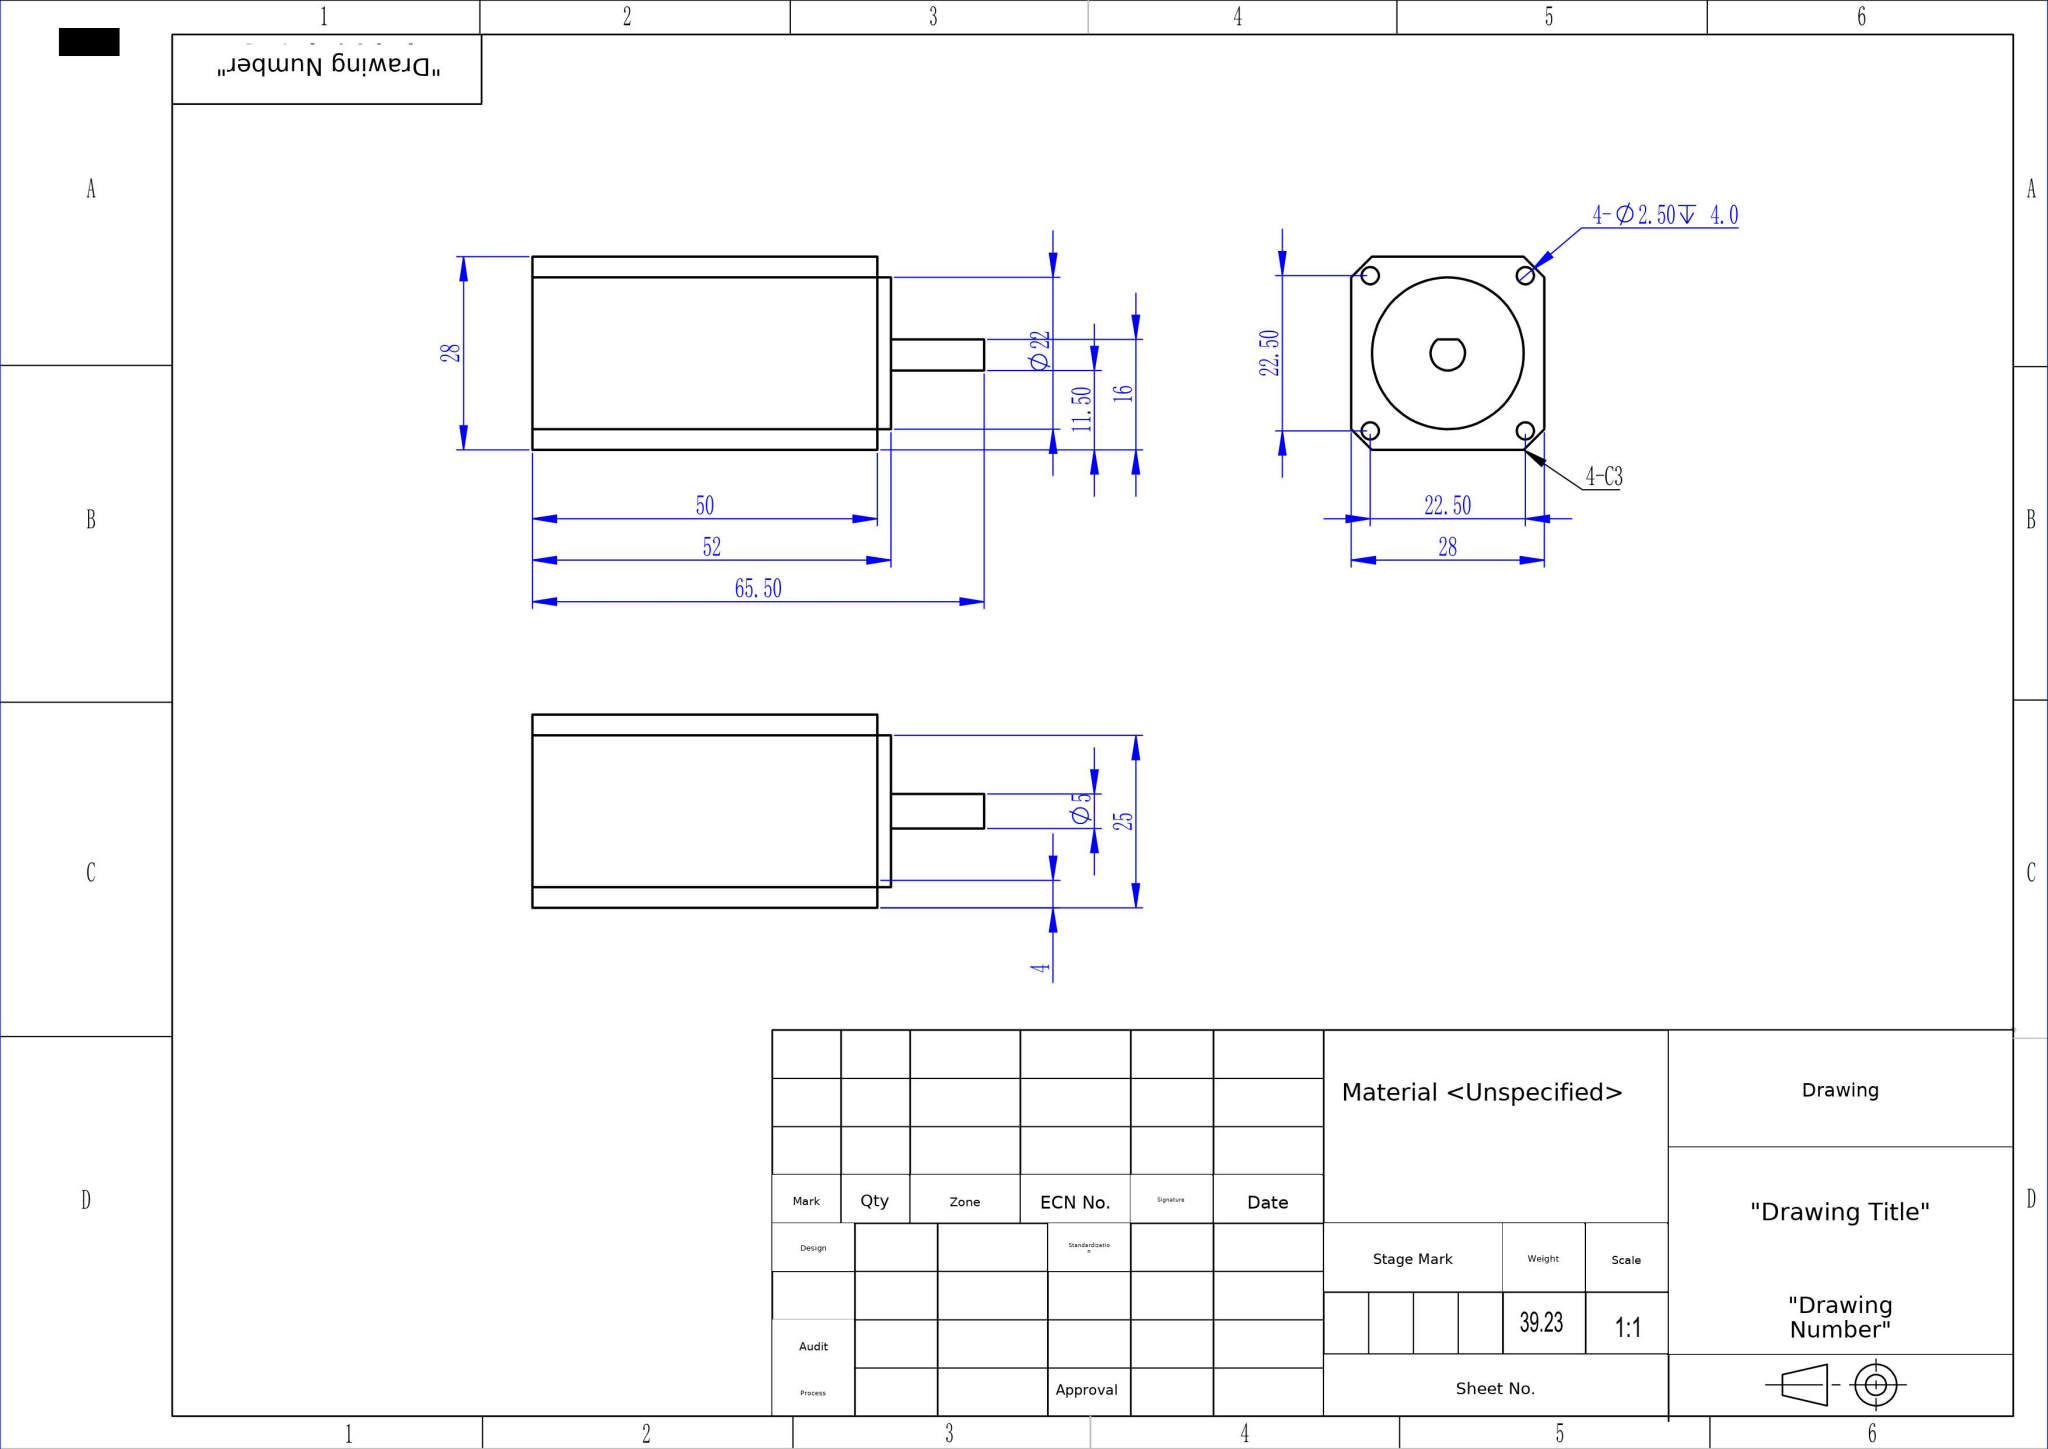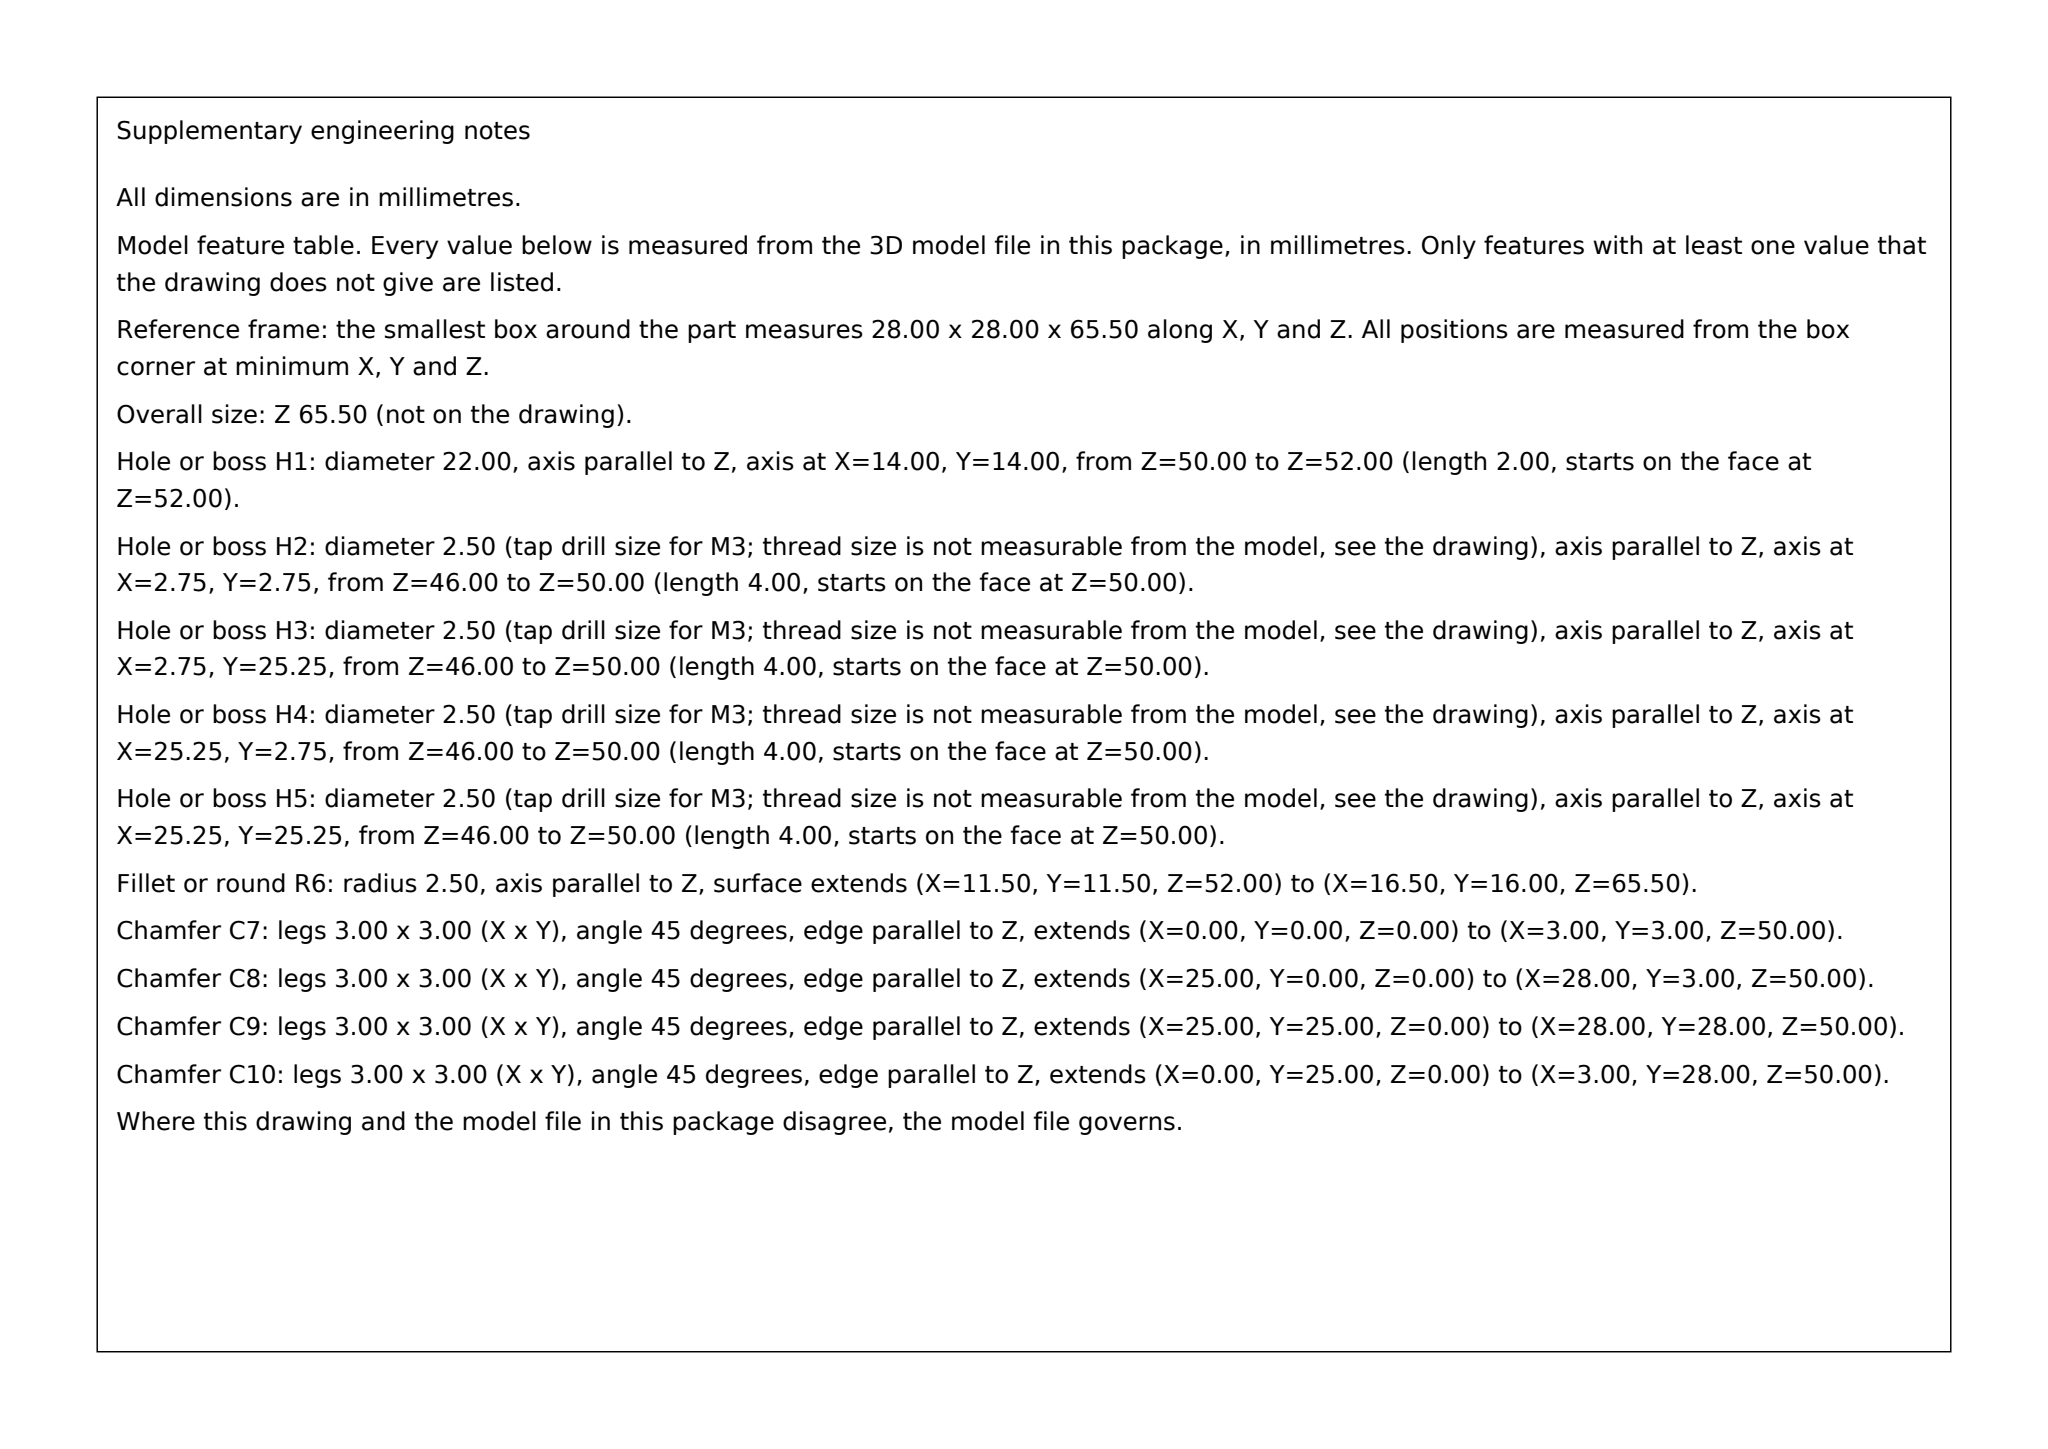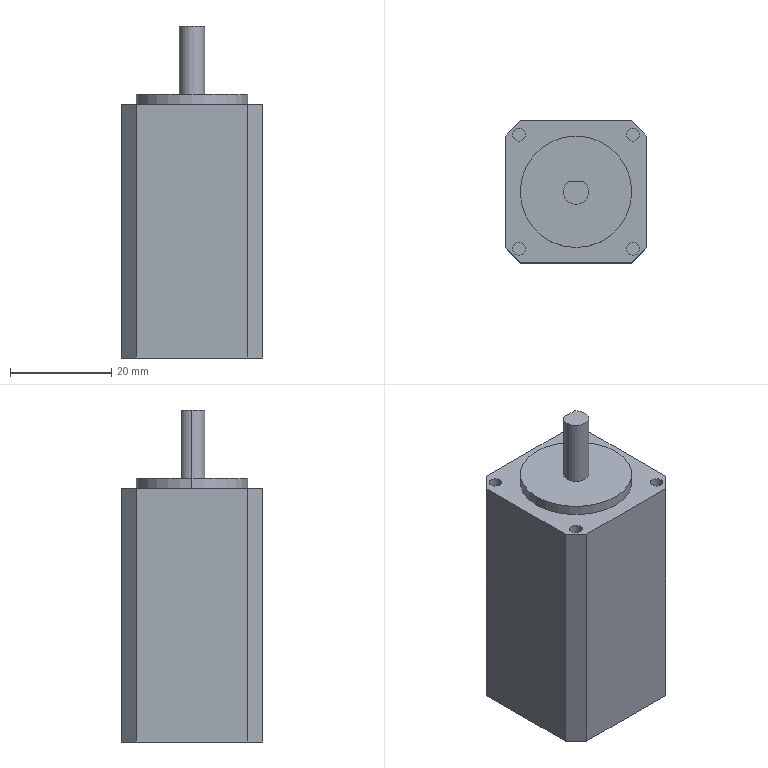Part | SolidWorks | mm | 1 solid | 30 faces | box 28 x 28 x 65.5 mm | volume 39233 mm3 | plane 17 | cylinder 13 | commonest cylinder face diameters 2.5 x8 5 x3 22 x2
build123d program:
from build123d import *

# Parameters (mm, degrees)
SKETCH1_W           = 28
SKETCH1_H           = 28
BOSS_EXTRUDE1_DEPTH = 50
SKETCH2_R           = 11
BOSS_EXTRUDE2_DEPTH = 2
SKETCH3_R           = 2.5
BOSS_EXTRUDE3_DEPTH = 13.5
CUT_EXTRUDE1_START  = -13.5
CUT_EXTRUDE1_DEPTH  = 13.5
SKETCH5_R           = 1.25
CUT_EXTRUDE2_DEPTH  = 4
CHAMFER1_SIZE       = 3


with BuildPart() as part:
    # Sketch1 → Boss-Extrude1 (new body)
    with BuildSketch(Plane.XY):
        Rectangle(SKETCH1_W, SKETCH1_H)
    extrude(amount=BOSS_EXTRUDE1_DEPTH)

    # Sketch2 → Boss-Extrude2 (add)
    with BuildSketch(Plane.XY.offset(50)):
        Circle(SKETCH2_R)
    extrude(amount=BOSS_EXTRUDE2_DEPTH)

    # Sketch3 → Boss-Extrude3 (add)
    with BuildSketch(Plane.XY.offset(52)):
        Circle(SKETCH3_R)
    extrude(amount=BOSS_EXTRUDE3_DEPTH)

    # Sketch4 → Cut-Extrude1 (cut)
    with BuildSketch(Plane.XY.offset(65.5).offset(CUT_EXTRUDE1_START)):
        with BuildLine():
            Line((-1.5, 2), (1.5, 2))
            ThreePointArc((1.5, 2), (0, 2.5), (-1.5, 2))
        make_face()
    extrude(amount=CUT_EXTRUDE1_DEPTH, mode=Mode.SUBTRACT)

    # Sketch5 → Cut-Extrude2 (cut)
    with BuildSketch(Plane.XY.offset(50)):
        with Locations((-11.25, -11.25)):
            Circle(SKETCH5_R)
        with Locations((11.25, -11.25)):
            Circle(SKETCH5_R)
        with Locations((11.25, 11.25)):
            Circle(SKETCH5_R)
        with Locations((-11.25, 11.25)):
            Circle(SKETCH5_R)
    extrude(amount=-CUT_EXTRUDE2_DEPTH, mode=Mode.SUBTRACT)

    # Chamfer1
    chamfer1_edges = [part.edges().sort_by_distance(p)[0] for p in [
        (14, -14, 25),
        (-14, -14, 25),
        (-14, 14, 25),
        (14, 14, 25),
    ]]
    chamfer(chamfer1_edges, length=CHAMFER1_SIZE)


solid = part.part
STEP:
#1=CARTESIAN_POINT('',(-12.5,11.25,46.));
#2=VERTEX_POINT('',#1);
#3=CARTESIAN_POINT('',(-10.,11.25,46.));
#4=VERTEX_POINT('',#3);
#5=CARTESIAN_POINT('',(-11.25,11.25,46.));
#6=DIRECTION('',(0.,0.,1.));
#7=DIRECTION('',(1.,0.,0.));
#8=AXIS2_PLACEMENT_3D('',#5,#6,#7);
#9=CIRCLE('',#8,1.25);
#10=EDGE_CURVE('',#2,#4,#9,.T.);
#11=ORIENTED_EDGE('',*,*,#10,.F.);
#12=CARTESIAN_POINT('',(-12.5,11.25,50.));
#13=VERTEX_POINT('',#12);
#14=CARTESIAN_POINT('',(-12.5,11.25,46.));
#15=DIRECTION('',(0.,0.,1.));
#16=VECTOR('',#15,1000.);
#17=LINE('',#14,#16);
#18=EDGE_CURVE('',#2,#13,#17,.T.);
#19=ORIENTED_EDGE('',*,*,#18,.T.);
#20=CARTESIAN_POINT('',(-10.,11.25,50.));
#21=VERTEX_POINT('',#20);
#22=CARTESIAN_POINT('',(-11.25,11.25,50.));
#23=DIRECTION('',(0.,0.,1.));
#24=DIRECTION('',(1.,0.,0.));
#25=AXIS2_PLACEMENT_3D('',#22,#23,#24);
#26=CIRCLE('',#25,1.25);
#27=EDGE_CURVE('',#13,#21,#26,.T.);
#28=ORIENTED_EDGE('',*,*,#27,.T.);
#29=CARTESIAN_POINT('',(-10.,11.25,46.));
#30=DIRECTION('',(0.,0.,1.));
#31=VECTOR('',#30,1000.);
#32=LINE('',#29,#31);
#33=EDGE_CURVE('',#4,#21,#32,.T.);
#34=ORIENTED_EDGE('',*,*,#33,.F.);
#35=EDGE_LOOP('',(#11,#19,#28,#34));
#36=FACE_OUTER_BOUND('',#35,.T.);
#37=CARTESIAN_POINT('',(-11.25,11.25,46.));
#38=DIRECTION('',(0.,0.,1.));
#39=DIRECTION('',(1.,0.,0.));
#40=AXIS2_PLACEMENT_3D('',#37,#38,#39);
#41=CYLINDRICAL_SURFACE('',#40,1.25);
#42=ADVANCED_FACE('',(#36),#41,.F.);
#43=CARTESIAN_POINT('',(10.,11.25,46.));
#44=VERTEX_POINT('',#43);
#45=CARTESIAN_POINT('',(12.5,11.25,46.));
#46=VERTEX_POINT('',#45);
#47=CARTESIAN_POINT('',(11.25,11.25,46.));
#48=DIRECTION('',(0.,0.,1.));
#49=DIRECTION('',(1.,0.,0.));
#50=AXIS2_PLACEMENT_3D('',#47,#48,#49);
#51=CIRCLE('',#50,1.25);
#52=EDGE_CURVE('',#44,#46,#51,.T.);
#53=ORIENTED_EDGE('',*,*,#52,.F.);
#54=CARTESIAN_POINT('',(10.,11.25,50.));
#55=VERTEX_POINT('',#54);
#56=CARTESIAN_POINT('',(10.,11.25,46.));
#57=DIRECTION('',(0.,0.,1.));
#58=VECTOR('',#57,1000.);
#59=LINE('',#56,#58);
#60=EDGE_CURVE('',#44,#55,#59,.T.);
#61=ORIENTED_EDGE('',*,*,#60,.T.);
#62=CARTESIAN_POINT('',(12.5,11.25,50.));
#63=VERTEX_POINT('',#62);
#64=CARTESIAN_POINT('',(11.25,11.25,50.));
#65=DIRECTION('',(0.,0.,1.));
#66=DIRECTION('',(1.,0.,0.));
#67=AXIS2_PLACEMENT_3D('',#64,#65,#66);
#68=CIRCLE('',#67,1.25);
#69=EDGE_CURVE('',#55,#63,#68,.T.);
#70=ORIENTED_EDGE('',*,*,#69,.T.);
#71=CARTESIAN_POINT('',(12.5,11.25,46.));
#72=DIRECTION('',(0.,0.,1.));
#73=VECTOR('',#72,1000.);
#74=LINE('',#71,#73);
#75=EDGE_CURVE('',#46,#63,#74,.T.);
#76=ORIENTED_EDGE('',*,*,#75,.F.);
#77=EDGE_LOOP('',(#53,#61,#70,#76));
#78=FACE_OUTER_BOUND('',#77,.T.);
#79=CARTESIAN_POINT('',(11.25,11.25,46.));
#80=DIRECTION('',(0.,0.,1.));
#81=DIRECTION('',(1.,0.,0.));
#82=AXIS2_PLACEMENT_3D('',#79,#80,#81);
#83=CYLINDRICAL_SURFACE('',#82,1.25);
#84=ADVANCED_FACE('',(#78),#83,.F.);
#85=CARTESIAN_POINT('',(10.,-11.25,46.));
#86=VERTEX_POINT('',#85);
#87=CARTESIAN_POINT('',(12.5,-11.25,46.));
#88=VERTEX_POINT('',#87);
#89=CARTESIAN_POINT('',(11.25,-11.25,46.));
#90=DIRECTION('',(0.,0.,1.));
#91=DIRECTION('',(1.,0.,0.));
#92=AXIS2_PLACEMENT_3D('',#89,#90,#91);
#93=CIRCLE('',#92,1.25);
#94=EDGE_CURVE('',#86,#88,#93,.T.);
#95=ORIENTED_EDGE('',*,*,#94,.F.);
#96=CARTESIAN_POINT('',(10.,-11.25,50.));
#97=VERTEX_POINT('',#96);
#98=CARTESIAN_POINT('',(10.,-11.25,46.));
#99=DIRECTION('',(0.,0.,1.));
#100=VECTOR('',#99,1000.);
#101=LINE('',#98,#100);
#102=EDGE_CURVE('',#86,#97,#101,.T.);
#103=ORIENTED_EDGE('',*,*,#102,.T.);
#104=CARTESIAN_POINT('',(12.5,-11.25,50.));
#105=VERTEX_POINT('',#104);
#106=CARTESIAN_POINT('',(11.25,-11.25,50.));
#107=DIRECTION('',(0.,0.,1.));
#108=DIRECTION('',(1.,0.,0.));
#109=AXIS2_PLACEMENT_3D('',#106,#107,#108);
#110=CIRCLE('',#109,1.25);
#111=EDGE_CURVE('',#97,#105,#110,.T.);
#112=ORIENTED_EDGE('',*,*,#111,.T.);
#113=CARTESIAN_POINT('',(12.5,-11.25,46.));
#114=DIRECTION('',(0.,0.,1.));
#115=VECTOR('',#114,1000.);
#116=LINE('',#113,#115);
#117=EDGE_CURVE('',#88,#105,#116,.T.);
#118=ORIENTED_EDGE('',*,*,#117,.F.);
#119=EDGE_LOOP('',(#95,#103,#112,#118));
#120=FACE_OUTER_BOUND('',#119,.T.);
#121=CARTESIAN_POINT('',(11.25,-11.25,46.));
#122=DIRECTION('',(0.,0.,1.));
#123=DIRECTION('',(1.,0.,0.));
#124=AXIS2_PLACEMENT_3D('',#121,#122,#123);
#125=CYLINDRICAL_SURFACE('',#124,1.25);
#126=ADVANCED_FACE('',(#120),#125,.F.);
#127=CARTESIAN_POINT('',(-12.5,-11.25,46.));
#128=VERTEX_POINT('',#127);
#129=CARTESIAN_POINT('',(-10.,-11.25,46.));
#130=VERTEX_POINT('',#129);
#131=CARTESIAN_POINT('',(-11.25,-11.25,46.));
#132=DIRECTION('',(0.,0.,1.));
#133=DIRECTION('',(1.,0.,0.));
#134=AXIS2_PLACEMENT_3D('',#131,#132,#133);
#135=CIRCLE('',#134,1.25);
#136=EDGE_CURVE('',#128,#130,#135,.T.);
#137=ORIENTED_EDGE('',*,*,#136,.F.);
#138=CARTESIAN_POINT('',(-12.5,-11.25,50.));
#139=VERTEX_POINT('',#138);
#140=CARTESIAN_POINT('',(-12.5,-11.25,46.));
#141=DIRECTION('',(0.,0.,1.));
#142=VECTOR('',#141,1000.);
#143=LINE('',#140,#142);
#144=EDGE_CURVE('',#128,#139,#143,.T.);
#145=ORIENTED_EDGE('',*,*,#144,.T.);
#146=CARTESIAN_POINT('',(-10.,-11.25,50.));
#147=VERTEX_POINT('',#146);
#148=CARTESIAN_POINT('',(-11.25,-11.25,50.));
#149=DIRECTION('',(0.,0.,1.));
#150=DIRECTION('',(1.,0.,0.));
#151=AXIS2_PLACEMENT_3D('',#148,#149,#150);
#152=CIRCLE('',#151,1.25);
#153=EDGE_CURVE('',#139,#147,#152,.T.);
#154=ORIENTED_EDGE('',*,*,#153,.T.);
#155=CARTESIAN_POINT('',(-10.,-11.25,46.));
#156=DIRECTION('',(0.,0.,1.));
#157=VECTOR('',#156,1000.);
#158=LINE('',#155,#157);
#159=EDGE_CURVE('',#130,#147,#158,.T.);
#160=ORIENTED_EDGE('',*,*,#159,.F.);
#161=EDGE_LOOP('',(#137,#145,#154,#160));
#162=FACE_OUTER_BOUND('',#161,.T.);
#163=CARTESIAN_POINT('',(-11.25,-11.25,46.));
#164=DIRECTION('',(0.,0.,1.));
#165=DIRECTION('',(1.,0.,0.));
#166=AXIS2_PLACEMENT_3D('',#163,#164,#165);
#167=CYLINDRICAL_SURFACE('',#166,1.25);
#168=ADVANCED_FACE('',(#162),#167,.F.);
#169=CARTESIAN_POINT('',(2.5,0.,65.5));
#170=VERTEX_POINT('',#169);
#171=CARTESIAN_POINT('',(1.5,2.,65.5));
#172=VERTEX_POINT('',#171);
#173=CARTESIAN_POINT('',(0.,0.,65.5));
#174=DIRECTION('',(0.,0.,1.));
#175=DIRECTION('',(1.,0.,0.));
#176=AXIS2_PLACEMENT_3D('',#173,#174,#175);
#177=CIRCLE('',#176,2.5);
#178=EDGE_CURVE('',#170,#172,#177,.T.);
#179=ORIENTED_EDGE('',*,*,#178,.F.);
#180=CARTESIAN_POINT('',(2.5,0.,52.));
#181=VERTEX_POINT('',#180);
#182=CARTESIAN_POINT('',(2.5,0.,65.5));
#183=DIRECTION('',(0.,0.,-1.));
#184=VECTOR('',#183,1000.);
#185=LINE('',#182,#184);
#186=EDGE_CURVE('',#170,#181,#185,.T.);
#187=ORIENTED_EDGE('',*,*,#186,.T.);
#188=CARTESIAN_POINT('',(1.5,2.,52.));
#189=VERTEX_POINT('',#188);
#190=CARTESIAN_POINT('',(0.,0.,52.));
#191=DIRECTION('',(0.,0.,1.));
#192=DIRECTION('',(1.,0.,0.));
#193=AXIS2_PLACEMENT_3D('',#190,#191,#192);
#194=CIRCLE('',#193,2.5);
#195=EDGE_CURVE('',#181,#189,#194,.T.);
#196=ORIENTED_EDGE('',*,*,#195,.T.);
#197=CARTESIAN_POINT('',(1.5,2.,52.));
#198=DIRECTION('',(0.,0.,1.));
#199=VECTOR('',#198,1000.);
#200=LINE('',#197,#199);
#201=EDGE_CURVE('',#189,#172,#200,.T.);
#202=ORIENTED_EDGE('',*,*,#201,.T.);
#203=EDGE_LOOP('',(#179,#187,#196,#202));
#204=FACE_OUTER_BOUND('',#203,.T.);
#205=CARTESIAN_POINT('',(0.,0.,65.5));
#206=DIRECTION('',(0.,0.,-1.));
#207=DIRECTION('',(-1.,0.,0.));
#208=AXIS2_PLACEMENT_3D('',#205,#206,#207);
#209=CYLINDRICAL_SURFACE('',#208,2.5);
#210=ADVANCED_FACE('',(#204),#209,.T.);
#211=ORIENTED_EDGE('',*,*,#186,.F.);
#212=CARTESIAN_POINT('',(-2.5,0.,65.5));
#213=VERTEX_POINT('',#212);
#214=CARTESIAN_POINT('',(0.,0.,65.5));
#215=DIRECTION('',(0.,0.,1.));
#216=DIRECTION('',(1.,0.,0.));
#217=AXIS2_PLACEMENT_3D('',#214,#215,#216);
#218=CIRCLE('',#217,2.5);
#219=EDGE_CURVE('',#213,#170,#218,.T.);
#220=ORIENTED_EDGE('',*,*,#219,.F.);
#221=CARTESIAN_POINT('',(-2.5,0.,52.));
#222=VERTEX_POINT('',#221);
#223=CARTESIAN_POINT('',(-2.5,0.,65.5));
#224=DIRECTION('',(0.,0.,-1.));
#225=VECTOR('',#224,1000.);
#226=LINE('',#223,#225);
#227=EDGE_CURVE('',#213,#222,#226,.T.);
#228=ORIENTED_EDGE('',*,*,#227,.T.);
#229=CARTESIAN_POINT('',(0.,0.,52.));
#230=DIRECTION('',(0.,0.,1.));
#231=DIRECTION('',(1.,0.,0.));
#232=AXIS2_PLACEMENT_3D('',#229,#230,#231);
#233=CIRCLE('',#232,2.5);
#234=EDGE_CURVE('',#222,#181,#233,.T.);
#235=ORIENTED_EDGE('',*,*,#234,.T.);
#236=EDGE_LOOP('',(#211,#220,#228,#235));
#237=FACE_OUTER_BOUND('',#236,.T.);
#238=CARTESIAN_POINT('',(0.,0.,65.5));
#239=DIRECTION('',(0.,0.,-1.));
#240=DIRECTION('',(-1.,0.,0.));
#241=AXIS2_PLACEMENT_3D('',#238,#239,#240);
#242=CYLINDRICAL_SURFACE('',#241,2.5);
#243=ADVANCED_FACE('',(#237),#242,.T.);
#244=CARTESIAN_POINT('',(11.,0.,52.));
#245=VERTEX_POINT('',#244);
#246=CARTESIAN_POINT('',(-11.,0.,52.));
#247=VERTEX_POINT('',#246);
#248=CARTESIAN_POINT('',(0.,0.,52.));
#249=DIRECTION('',(0.,0.,1.));
#250=DIRECTION('',(1.,0.,0.));
#251=AXIS2_PLACEMENT_3D('',#248,#249,#250);
#252=CIRCLE('',#251,11.);
#253=EDGE_CURVE('',#245,#247,#252,.T.);
#254=ORIENTED_EDGE('',*,*,#253,.F.);
#255=CARTESIAN_POINT('',(11.,0.,50.));
#256=VERTEX_POINT('',#255);
#257=CARTESIAN_POINT('',(11.,0.,52.));
#258=DIRECTION('',(0.,0.,-1.));
#259=VECTOR('',#258,1000.);
#260=LINE('',#257,#259);
#261=EDGE_CURVE('',#245,#256,#260,.T.);
#262=ORIENTED_EDGE('',*,*,#261,.T.);
#263=CARTESIAN_POINT('',(-11.,0.,50.));
#264=VERTEX_POINT('',#263);
#265=CARTESIAN_POINT('',(0.,0.,50.));
#266=DIRECTION('',(0.,0.,1.));
#267=DIRECTION('',(1.,0.,0.));
#268=AXIS2_PLACEMENT_3D('',#265,#266,#267);
#269=CIRCLE('',#268,11.);
#270=EDGE_CURVE('',#256,#264,#269,.T.);
#271=ORIENTED_EDGE('',*,*,#270,.T.);
#272=CARTESIAN_POINT('',(-11.,0.,52.));
#273=DIRECTION('',(0.,0.,-1.));
#274=VECTOR('',#273,1000.);
#275=LINE('',#272,#274);
#276=EDGE_CURVE('',#247,#264,#275,.T.);
#277=ORIENTED_EDGE('',*,*,#276,.F.);
#278=EDGE_LOOP('',(#254,#262,#271,#277));
#279=FACE_OUTER_BOUND('',#278,.T.);
#280=CARTESIAN_POINT('',(0.,0.,52.));
#281=DIRECTION('',(0.,0.,-1.));
#282=DIRECTION('',(-1.,0.,0.));
#283=AXIS2_PLACEMENT_3D('',#280,#281,#282);
#284=CYLINDRICAL_SURFACE('',#283,11.);
#285=ADVANCED_FACE('',(#279),#284,.T.);
#286=CARTESIAN_POINT('',(14.,-11.,50.));
#287=VERTEX_POINT('',#286);
#288=CARTESIAN_POINT('',(14.,11.,50.));
#289=VERTEX_POINT('',#288);
#290=CARTESIAN_POINT('',(14.,14.,50.));
#291=DIRECTION('',(-0.,1.,0.));
#292=VECTOR('',#291,1000.);
#293=LINE('',#290,#292);
#294=EDGE_CURVE('',#287,#289,#293,.T.);
#295=ORIENTED_EDGE('',*,*,#294,.F.);
#296=CARTESIAN_POINT('',(14.,-11.,0.));
#297=VERTEX_POINT('',#296);
#298=CARTESIAN_POINT('',(14.,-11.,50.));
#299=DIRECTION('',(0.,0.,-1.));
#300=VECTOR('',#299,1000.);
#301=LINE('',#298,#300);
#302=EDGE_CURVE('',#287,#297,#301,.T.);
#303=ORIENTED_EDGE('',*,*,#302,.T.);
#304=CARTESIAN_POINT('',(14.,11.,0.));
#305=VERTEX_POINT('',#304);
#306=CARTESIAN_POINT('',(14.,14.,0.));
#307=DIRECTION('',(-0.,1.,0.));
#308=VECTOR('',#307,1000.);
#309=LINE('',#306,#308);
#310=EDGE_CURVE('',#297,#305,#309,.T.);
#311=ORIENTED_EDGE('',*,*,#310,.T.);
#312=CARTESIAN_POINT('',(14.,11.,50.));
#313=DIRECTION('',(0.,0.,1.));
#314=VECTOR('',#313,1000.);
#315=LINE('',#312,#314);
#316=EDGE_CURVE('',#305,#289,#315,.T.);
#317=ORIENTED_EDGE('',*,*,#316,.T.);
#318=EDGE_LOOP('',(#295,#303,#311,#317));
#319=FACE_OUTER_BOUND('',#318,.T.);
#320=CARTESIAN_POINT('',(14.,14.,50.));
#321=DIRECTION('',(-1.,-0.,0.));
#322=DIRECTION('',(0.,-1.,0.));
#323=AXIS2_PLACEMENT_3D('',#320,#321,#322);
#324=PLANE('',#323);
#325=ADVANCED_FACE('',(#319),#324,.F.);
#326=CARTESIAN_POINT('',(11.,14.,50.));
#327=VERTEX_POINT('',#326);
#328=CARTESIAN_POINT('',(-11.,14.,50.));
#329=VERTEX_POINT('',#328);
#330=CARTESIAN_POINT('',(-14.,14.,50.));
#331=DIRECTION('',(-1.,0.,0.));
#332=VECTOR('',#331,1000.);
#333=LINE('',#330,#332);
#334=EDGE_CURVE('',#327,#329,#333,.T.);
#335=ORIENTED_EDGE('',*,*,#334,.F.);
#336=CARTESIAN_POINT('',(11.,14.,0.));
#337=VERTEX_POINT('',#336);
#338=CARTESIAN_POINT('',(11.,14.,50.));
#339=DIRECTION('',(0.,0.,-1.));
#340=VECTOR('',#339,1000.);
#341=LINE('',#338,#340);
#342=EDGE_CURVE('',#327,#337,#341,.T.);
#343=ORIENTED_EDGE('',*,*,#342,.T.);
#344=CARTESIAN_POINT('',(-11.,14.,0.));
#345=VERTEX_POINT('',#344);
#346=CARTESIAN_POINT('',(-14.,14.,0.));
#347=DIRECTION('',(-1.,0.,0.));
#348=VECTOR('',#347,1000.);
#349=LINE('',#346,#348);
#350=EDGE_CURVE('',#337,#345,#349,.T.);
#351=ORIENTED_EDGE('',*,*,#350,.T.);
#352=CARTESIAN_POINT('',(-11.,14.,50.));
#353=DIRECTION('',(0.,0.,1.));
#354=VECTOR('',#353,1000.);
#355=LINE('',#352,#354);
#356=EDGE_CURVE('',#345,#329,#355,.T.);
#357=ORIENTED_EDGE('',*,*,#356,.T.);
#358=EDGE_LOOP('',(#335,#343,#351,#357));
#359=FACE_OUTER_BOUND('',#358,.T.);
#360=CARTESIAN_POINT('',(-14.,14.,50.));
#361=DIRECTION('',(0.,-1.,0.));
#362=DIRECTION('',(0.,0.,-1.));
#363=AXIS2_PLACEMENT_3D('',#360,#361,#362);
#364=PLANE('',#363);
#365=ADVANCED_FACE('',(#359),#364,.F.);
#366=CARTESIAN_POINT('',(-14.,11.,0.));
#367=VERTEX_POINT('',#366);
#368=CARTESIAN_POINT('',(-14.,-11.,0.));
#369=VERTEX_POINT('',#368);
#370=CARTESIAN_POINT('',(-14.,14.,0.));
#371=DIRECTION('',(0.,-1.,0.));
#372=VECTOR('',#371,1000.);
#373=LINE('',#370,#372);
#374=EDGE_CURVE('',#367,#369,#373,.T.);
#375=ORIENTED_EDGE('',*,*,#374,.T.);
#376=CARTESIAN_POINT('',(-14.,-11.,50.));
#377=VERTEX_POINT('',#376);
#378=CARTESIAN_POINT('',(-14.,-11.,50.));
#379=DIRECTION('',(0.,0.,1.));
#380=VECTOR('',#379,1000.);
#381=LINE('',#378,#380);
#382=EDGE_CURVE('',#369,#377,#381,.T.);
#383=ORIENTED_EDGE('',*,*,#382,.T.);
#384=CARTESIAN_POINT('',(-14.,11.,50.));
#385=VERTEX_POINT('',#384);
#386=CARTESIAN_POINT('',(-14.,14.,50.));
#387=DIRECTION('',(0.,-1.,0.));
#388=VECTOR('',#387,1000.);
#389=LINE('',#386,#388);
#390=EDGE_CURVE('',#385,#377,#389,.T.);
#391=ORIENTED_EDGE('',*,*,#390,.F.);
#392=CARTESIAN_POINT('',(-14.,11.,50.));
#393=DIRECTION('',(0.,0.,-1.));
#394=VECTOR('',#393,1000.);
#395=LINE('',#392,#394);
#396=EDGE_CURVE('',#385,#367,#395,.T.);
#397=ORIENTED_EDGE('',*,*,#396,.T.);
#398=EDGE_LOOP('',(#375,#383,#391,#397));
#399=FACE_OUTER_BOUND('',#398,.T.);
#400=CARTESIAN_POINT('',(-14.,14.,50.));
#401=DIRECTION('',(1.,0.,0.));
#402=DIRECTION('',(-0.,1.,0.));
#403=AXIS2_PLACEMENT_3D('',#400,#401,#402);
#404=PLANE('',#403);
#405=ADVANCED_FACE('',(#399),#404,.F.);
#406=CARTESIAN_POINT('',(-11.,-14.,50.));
#407=VERTEX_POINT('',#406);
#408=CARTESIAN_POINT('',(11.,-14.,50.));
#409=VERTEX_POINT('',#408);
#410=CARTESIAN_POINT('',(-14.,-14.,50.));
#411=DIRECTION('',(1.,0.,0.));
#412=VECTOR('',#411,1000.);
#413=LINE('',#410,#412);
#414=EDGE_CURVE('',#407,#409,#413,.T.);
#415=ORIENTED_EDGE('',*,*,#414,.F.);
#416=CARTESIAN_POINT('',(-11.,-14.,0.));
#417=VERTEX_POINT('',#416);
#418=CARTESIAN_POINT('',(-11.,-14.,50.));
#419=DIRECTION('',(0.,0.,-1.));
#420=VECTOR('',#419,1000.);
#421=LINE('',#418,#420);
#422=EDGE_CURVE('',#407,#417,#421,.T.);
#423=ORIENTED_EDGE('',*,*,#422,.T.);
#424=CARTESIAN_POINT('',(11.,-14.,0.));
#425=VERTEX_POINT('',#424);
#426=CARTESIAN_POINT('',(-14.,-14.,0.));
#427=DIRECTION('',(1.,0.,0.));
#428=VECTOR('',#427,1000.);
#429=LINE('',#426,#428);
#430=EDGE_CURVE('',#417,#425,#429,.T.);
#431=ORIENTED_EDGE('',*,*,#430,.T.);
#432=CARTESIAN_POINT('',(11.,-14.,50.));
#433=DIRECTION('',(0.,0.,1.));
#434=VECTOR('',#433,1000.);
#435=LINE('',#432,#434);
#436=EDGE_CURVE('',#425,#409,#435,.T.);
#437=ORIENTED_EDGE('',*,*,#436,.T.);
#438=EDGE_LOOP('',(#415,#423,#431,#437));
#439=FACE_OUTER_BOUND('',#438,.T.);
#440=CARTESIAN_POINT('',(-14.,-14.,50.));
#441=DIRECTION('',(0.,1.,0.));
#442=DIRECTION('',(0.,0.,1.));
#443=AXIS2_PLACEMENT_3D('',#440,#441,#442);
#444=PLANE('',#443);
#445=ADVANCED_FACE('',(#439),#444,.F.);
#446=CARTESIAN_POINT('',(-11.25,11.25,50.));
#447=DIRECTION('',(0.,0.,1.));
#448=DIRECTION('',(1.,0.,0.));
#449=AXIS2_PLACEMENT_3D('',#446,#447,#448);
#450=CIRCLE('',#449,1.25);
#451=EDGE_CURVE('',#21,#13,#450,.T.);
#452=ORIENTED_EDGE('',*,*,#451,.F.);
#453=ORIENTED_EDGE('',*,*,#27,.F.);
#454=EDGE_LOOP('',(#452,#453));
#455=FACE_BOUND('',#454,.T.);
#456=CARTESIAN_POINT('',(11.25,11.25,50.));
#457=DIRECTION('',(0.,0.,1.));
#458=DIRECTION('',(1.,0.,0.));
#459=AXIS2_PLACEMENT_3D('',#456,#457,#458);
#460=CIRCLE('',#459,1.25);
#461=EDGE_CURVE('',#63,#55,#460,.T.);
#462=ORIENTED_EDGE('',*,*,#461,.F.);
#463=ORIENTED_EDGE('',*,*,#69,.F.);
#464=EDGE_LOOP('',(#462,#463));
#465=FACE_BOUND('',#464,.T.);
#466=CARTESIAN_POINT('',(11.25,-11.25,50.));
#467=DIRECTION('',(0.,0.,1.));
#468=DIRECTION('',(1.,0.,0.));
#469=AXIS2_PLACEMENT_3D('',#466,#467,#468);
#470=CIRCLE('',#469,1.25);
#471=EDGE_CURVE('',#105,#97,#470,.T.);
#472=ORIENTED_EDGE('',*,*,#471,.F.);
#473=ORIENTED_EDGE('',*,*,#111,.F.);
#474=EDGE_LOOP('',(#472,#473));
#475=FACE_BOUND('',#474,.T.);
#476=CARTESIAN_POINT('',(-11.25,-11.25,50.));
#477=DIRECTION('',(0.,0.,1.));
#478=DIRECTION('',(1.,0.,0.));
#479=AXIS2_PLACEMENT_3D('',#476,#477,#478);
#480=CIRCLE('',#479,1.25);
#481=EDGE_CURVE('',#147,#139,#480,.T.);
#482=ORIENTED_EDGE('',*,*,#481,.F.);
#483=ORIENTED_EDGE('',*,*,#153,.F.);
#484=EDGE_LOOP('',(#482,#483));
#485=FACE_BOUND('',#484,.T.);
#486=CARTESIAN_POINT('',(0.,0.,50.));
#487=DIRECTION('',(0.,0.,1.));
#488=DIRECTION('',(1.,0.,0.));
#489=AXIS2_PLACEMENT_3D('',#486,#487,#488);
#490=CIRCLE('',#489,11.);
#491=EDGE_CURVE('',#264,#256,#490,.T.);
#492=ORIENTED_EDGE('',*,*,#491,.F.);
#493=ORIENTED_EDGE('',*,*,#270,.F.);
#494=EDGE_LOOP('',(#492,#493));
#495=FACE_BOUND('',#494,.T.);
#496=ORIENTED_EDGE('',*,*,#390,.T.);
#497=CARTESIAN_POINT('',(-12.5,-12.5,50.));
#498=DIRECTION('',(0.7071,-0.7071,0.));
#499=VECTOR('',#498,1000.);
#500=LINE('',#497,#499);
#501=EDGE_CURVE('',#377,#407,#500,.T.);
#502=ORIENTED_EDGE('',*,*,#501,.T.);
#503=ORIENTED_EDGE('',*,*,#414,.T.);
#504=CARTESIAN_POINT('',(12.5,-12.5,50.));
#505=DIRECTION('',(0.7071,0.7071,0.));
#506=VECTOR('',#505,1000.);
#507=LINE('',#504,#506);
#508=EDGE_CURVE('',#409,#287,#507,.T.);
#509=ORIENTED_EDGE('',*,*,#508,.T.);
#510=ORIENTED_EDGE('',*,*,#294,.T.);
#511=CARTESIAN_POINT('',(12.5,12.5,50.));
#512=DIRECTION('',(-0.7071,0.7071,0.));
#513=VECTOR('',#512,1000.);
#514=LINE('',#511,#513);
#515=EDGE_CURVE('',#289,#327,#514,.T.);
#516=ORIENTED_EDGE('',*,*,#515,.T.);
#517=ORIENTED_EDGE('',*,*,#334,.T.);
#518=CARTESIAN_POINT('',(-12.5,12.5,50.));
#519=DIRECTION('',(-0.7071,-0.7071,0.));
#520=VECTOR('',#519,1000.);
#521=LINE('',#518,#520);
#522=EDGE_CURVE('',#329,#385,#521,.T.);
#523=ORIENTED_EDGE('',*,*,#522,.T.);
#524=EDGE_LOOP('',(#496,#502,#503,#509,#510,#516,#517,#523));
#525=FACE_OUTER_BOUND('',#524,.T.);
#526=CARTESIAN_POINT('',(0.,0.,50.));
#527=DIRECTION('',(0.,0.,1.));
#528=DIRECTION('',(1.,0.,0.));
#529=AXIS2_PLACEMENT_3D('',#526,#527,#528);
#530=PLANE('',#529);
#531=ADVANCED_FACE('',(#455,#465,#475,#485,#495,#525),#530,.T.);
#532=ORIENTED_EDGE('',*,*,#430,.F.);
#533=CARTESIAN_POINT('',(-11.,-14.,0.));
#534=DIRECTION('',(-0.7071,0.7071,0.));
#535=VECTOR('',#534,1000.);
#536=LINE('',#533,#535);
#537=EDGE_CURVE('',#417,#369,#536,.T.);
#538=ORIENTED_EDGE('',*,*,#537,.T.);
#539=ORIENTED_EDGE('',*,*,#374,.F.);
#540=CARTESIAN_POINT('',(-14.,11.,0.));
#541=DIRECTION('',(0.7071,0.7071,0.));
#542=VECTOR('',#541,1000.);
#543=LINE('',#540,#542);
#544=EDGE_CURVE('',#367,#345,#543,.T.);
#545=ORIENTED_EDGE('',*,*,#544,.T.);
#546=ORIENTED_EDGE('',*,*,#350,.F.);
#547=CARTESIAN_POINT('',(11.,14.,0.));
#548=DIRECTION('',(0.7071,-0.7071,0.));
#549=VECTOR('',#548,1000.);
#550=LINE('',#547,#549);
#551=EDGE_CURVE('',#337,#305,#550,.T.);
#552=ORIENTED_EDGE('',*,*,#551,.T.);
#553=ORIENTED_EDGE('',*,*,#310,.F.);
#554=CARTESIAN_POINT('',(14.,-11.,0.));
#555=DIRECTION('',(-0.7071,-0.7071,0.));
#556=VECTOR('',#555,1000.);
#557=LINE('',#554,#556);
#558=EDGE_CURVE('',#297,#425,#557,.T.);
#559=ORIENTED_EDGE('',*,*,#558,.T.);
#560=EDGE_LOOP('',(#532,#538,#539,#545,#546,#552,#553,#559));
#561=FACE_OUTER_BOUND('',#560,.T.);
#562=CARTESIAN_POINT('',(0.,0.,0.));
#563=DIRECTION('',(0.,0.,1.));
#564=DIRECTION('',(1.,0.,0.));
#565=AXIS2_PLACEMENT_3D('',#562,#563,#564);
#566=PLANE('',#565);
#567=ADVANCED_FACE('',(#561),#566,.F.);
#568=ORIENTED_EDGE('',*,*,#261,.F.);
#569=CARTESIAN_POINT('',(0.,0.,52.));
#570=DIRECTION('',(0.,0.,1.));
#571=DIRECTION('',(1.,0.,0.));
#572=AXIS2_PLACEMENT_3D('',#569,#570,#571);
#573=CIRCLE('',#572,11.);
#574=EDGE_CURVE('',#247,#245,#573,.T.);
#575=ORIENTED_EDGE('',*,*,#574,.F.);
#576=ORIENTED_EDGE('',*,*,#276,.T.);
#577=ORIENTED_EDGE('',*,*,#491,.T.);
#578=EDGE_LOOP('',(#568,#575,#576,#577));
#579=FACE_OUTER_BOUND('',#578,.T.);
#580=CARTESIAN_POINT('',(0.,0.,52.));
#581=DIRECTION('',(0.,0.,-1.));
#582=DIRECTION('',(-1.,0.,0.));
#583=AXIS2_PLACEMENT_3D('',#580,#581,#582);
#584=CYLINDRICAL_SURFACE('',#583,11.);
#585=ADVANCED_FACE('',(#579),#584,.T.);
#586=CARTESIAN_POINT('',(-1.5,2.,52.));
#587=VERTEX_POINT('',#586);
#588=CARTESIAN_POINT('',(0.,0.,52.));
#589=DIRECTION('',(0.,0.,1.));
#590=DIRECTION('',(1.,0.,0.));
#591=AXIS2_PLACEMENT_3D('',#588,#589,#590);
#592=CIRCLE('',#591,2.5);
#593=EDGE_CURVE('',#587,#222,#592,.T.);
#594=ORIENTED_EDGE('',*,*,#593,.F.);
#595=CARTESIAN_POINT('',(-1.5,2.,52.));
#596=DIRECTION('',(1.,0.,0.));
#597=VECTOR('',#596,1000.);
#598=LINE('',#595,#597);
#599=EDGE_CURVE('',#587,#189,#598,.T.);
#600=ORIENTED_EDGE('',*,*,#599,.T.);
#601=ORIENTED_EDGE('',*,*,#195,.F.);
#602=ORIENTED_EDGE('',*,*,#234,.F.);
#603=EDGE_LOOP('',(#594,#600,#601,#602));
#604=FACE_BOUND('',#603,.T.);
#605=ORIENTED_EDGE('',*,*,#574,.T.);
#606=ORIENTED_EDGE('',*,*,#253,.T.);
#607=EDGE_LOOP('',(#605,#606));
#608=FACE_OUTER_BOUND('',#607,.T.);
#609=CARTESIAN_POINT('',(0.,0.,52.));
#610=DIRECTION('',(0.,0.,1.));
#611=DIRECTION('',(1.,0.,0.));
#612=AXIS2_PLACEMENT_3D('',#609,#610,#611);
#613=PLANE('',#612);
#614=ADVANCED_FACE('',(#604,#608),#613,.T.);
#615=ORIENTED_EDGE('',*,*,#227,.F.);
#616=CARTESIAN_POINT('',(-1.5,2.,65.5));
#617=VERTEX_POINT('',#616);
#618=CARTESIAN_POINT('',(0.,0.,65.5));
#619=DIRECTION('',(0.,0.,1.));
#620=DIRECTION('',(1.,0.,0.));
#621=AXIS2_PLACEMENT_3D('',#618,#619,#620);
#622=CIRCLE('',#621,2.5);
#623=EDGE_CURVE('',#617,#213,#622,.T.);
#624=ORIENTED_EDGE('',*,*,#623,.F.);
#625=CARTESIAN_POINT('',(-1.5,2.,52.));
#626=DIRECTION('',(0.,0.,1.));
#627=VECTOR('',#626,1000.);
#628=LINE('',#625,#627);
#629=EDGE_CURVE('',#587,#617,#628,.T.);
#630=ORIENTED_EDGE('',*,*,#629,.F.);
#631=ORIENTED_EDGE('',*,*,#593,.T.);
#632=EDGE_LOOP('',(#615,#624,#630,#631));
#633=FACE_OUTER_BOUND('',#632,.T.);
#634=CARTESIAN_POINT('',(0.,0.,65.5));
#635=DIRECTION('',(0.,0.,-1.));
#636=DIRECTION('',(-1.,0.,0.));
#637=AXIS2_PLACEMENT_3D('',#634,#635,#636);
#638=CYLINDRICAL_SURFACE('',#637,2.5);
#639=ADVANCED_FACE('',(#633),#638,.T.);
#640=CARTESIAN_POINT('',(-1.5,2.,65.5));
#641=DIRECTION('',(1.,0.,0.));
#642=VECTOR('',#641,1000.);
#643=LINE('',#640,#642);
#644=EDGE_CURVE('',#617,#172,#643,.T.);
#645=ORIENTED_EDGE('',*,*,#644,.F.);
#646=ORIENTED_EDGE('',*,*,#623,.T.);
#647=ORIENTED_EDGE('',*,*,#219,.T.);
#648=ORIENTED_EDGE('',*,*,#178,.T.);
#649=EDGE_LOOP('',(#645,#646,#647,#648));
#650=FACE_OUTER_BOUND('',#649,.T.);
#651=CARTESIAN_POINT('',(0.,0.,65.5));
#652=DIRECTION('',(0.,0.,1.));
#653=DIRECTION('',(1.,0.,0.));
#654=AXIS2_PLACEMENT_3D('',#651,#652,#653);
#655=PLANE('',#654);
#656=ADVANCED_FACE('',(#650),#655,.T.);
#657=ORIENTED_EDGE('',*,*,#644,.T.);
#658=ORIENTED_EDGE('',*,*,#201,.F.);
#659=ORIENTED_EDGE('',*,*,#599,.F.);
#660=ORIENTED_EDGE('',*,*,#629,.T.);
#661=EDGE_LOOP('',(#657,#658,#659,#660));
#662=FACE_OUTER_BOUND('',#661,.T.);
#663=CARTESIAN_POINT('',(-1.5,2.,52.));
#664=DIRECTION('',(0.,-1.,0.));
#665=DIRECTION('',(0.,0.,-1.));
#666=AXIS2_PLACEMENT_3D('',#663,#664,#665);
#667=PLANE('',#666);
#668=ADVANCED_FACE('',(#662),#667,.F.);
#669=ORIENTED_EDGE('',*,*,#144,.F.);
#670=CARTESIAN_POINT('',(-11.25,-11.25,46.));
#671=DIRECTION('',(0.,0.,1.));
#672=DIRECTION('',(1.,0.,0.));
#673=AXIS2_PLACEMENT_3D('',#670,#671,#672);
#674=CIRCLE('',#673,1.25);
#675=EDGE_CURVE('',#130,#128,#674,.T.);
#676=ORIENTED_EDGE('',*,*,#675,.F.);
#677=ORIENTED_EDGE('',*,*,#159,.T.);
#678=ORIENTED_EDGE('',*,*,#481,.T.);
#679=EDGE_LOOP('',(#669,#676,#677,#678));
#680=FACE_OUTER_BOUND('',#679,.T.);
#681=CARTESIAN_POINT('',(-11.25,-11.25,46.));
#682=DIRECTION('',(0.,0.,1.));
#683=DIRECTION('',(1.,0.,0.));
#684=AXIS2_PLACEMENT_3D('',#681,#682,#683);
#685=CYLINDRICAL_SURFACE('',#684,1.25);
#686=ADVANCED_FACE('',(#680),#685,.F.);
#687=ORIENTED_EDGE('',*,*,#675,.T.);
#688=ORIENTED_EDGE('',*,*,#136,.T.);
#689=EDGE_LOOP('',(#687,#688));
#690=FACE_OUTER_BOUND('',#689,.T.);
#691=CARTESIAN_POINT('',(-11.25,-11.25,46.));
#692=DIRECTION('',(0.,0.,1.));
#693=DIRECTION('',(1.,0.,0.));
#694=AXIS2_PLACEMENT_3D('',#691,#692,#693);
#695=PLANE('',#694);
#696=ADVANCED_FACE('',(#690),#695,.T.);
#697=ORIENTED_EDGE('',*,*,#102,.F.);
#698=CARTESIAN_POINT('',(11.25,-11.25,46.));
#699=DIRECTION('',(0.,0.,1.));
#700=DIRECTION('',(1.,0.,0.));
#701=AXIS2_PLACEMENT_3D('',#698,#699,#700);
#702=CIRCLE('',#701,1.25);
#703=EDGE_CURVE('',#88,#86,#702,.T.);
#704=ORIENTED_EDGE('',*,*,#703,.F.);
#705=ORIENTED_EDGE('',*,*,#117,.T.);
#706=ORIENTED_EDGE('',*,*,#471,.T.);
#707=EDGE_LOOP('',(#697,#704,#705,#706));
#708=FACE_OUTER_BOUND('',#707,.T.);
#709=CARTESIAN_POINT('',(11.25,-11.25,46.));
#710=DIRECTION('',(0.,0.,1.));
#711=DIRECTION('',(1.,0.,0.));
#712=AXIS2_PLACEMENT_3D('',#709,#710,#711);
#713=CYLINDRICAL_SURFACE('',#712,1.25);
#714=ADVANCED_FACE('',(#708),#713,.F.);
#715=ORIENTED_EDGE('',*,*,#703,.T.);
#716=ORIENTED_EDGE('',*,*,#94,.T.);
#717=EDGE_LOOP('',(#715,#716));
#718=FACE_OUTER_BOUND('',#717,.T.);
#719=CARTESIAN_POINT('',(11.25,-11.25,46.));
#720=DIRECTION('',(0.,0.,1.));
#721=DIRECTION('',(1.,0.,0.));
#722=AXIS2_PLACEMENT_3D('',#719,#720,#721);
#723=PLANE('',#722);
#724=ADVANCED_FACE('',(#718),#723,.T.);
#725=ORIENTED_EDGE('',*,*,#60,.F.);
#726=CARTESIAN_POINT('',(11.25,11.25,46.));
#727=DIRECTION('',(0.,0.,1.));
#728=DIRECTION('',(1.,0.,0.));
#729=AXIS2_PLACEMENT_3D('',#726,#727,#728);
#730=CIRCLE('',#729,1.25);
#731=EDGE_CURVE('',#46,#44,#730,.T.);
#732=ORIENTED_EDGE('',*,*,#731,.F.);
#733=ORIENTED_EDGE('',*,*,#75,.T.);
#734=ORIENTED_EDGE('',*,*,#461,.T.);
#735=EDGE_LOOP('',(#725,#732,#733,#734));
#736=FACE_OUTER_BOUND('',#735,.T.);
#737=CARTESIAN_POINT('',(11.25,11.25,46.));
#738=DIRECTION('',(0.,0.,1.));
#739=DIRECTION('',(1.,0.,0.));
#740=AXIS2_PLACEMENT_3D('',#737,#738,#739);
#741=CYLINDRICAL_SURFACE('',#740,1.25);
#742=ADVANCED_FACE('',(#736),#741,.F.);
#743=ORIENTED_EDGE('',*,*,#731,.T.);
#744=ORIENTED_EDGE('',*,*,#52,.T.);
#745=EDGE_LOOP('',(#743,#744));
#746=FACE_OUTER_BOUND('',#745,.T.);
#747=CARTESIAN_POINT('',(11.25,11.25,46.));
#748=DIRECTION('',(0.,0.,1.));
#749=DIRECTION('',(1.,0.,0.));
#750=AXIS2_PLACEMENT_3D('',#747,#748,#749);
#751=PLANE('',#750);
#752=ADVANCED_FACE('',(#746),#751,.T.);
#753=ORIENTED_EDGE('',*,*,#18,.F.);
#754=CARTESIAN_POINT('',(-11.25,11.25,46.));
#755=DIRECTION('',(0.,0.,1.));
#756=DIRECTION('',(1.,0.,0.));
#757=AXIS2_PLACEMENT_3D('',#754,#755,#756);
#758=CIRCLE('',#757,1.25);
#759=EDGE_CURVE('',#4,#2,#758,.T.);
#760=ORIENTED_EDGE('',*,*,#759,.F.);
#761=ORIENTED_EDGE('',*,*,#33,.T.);
#762=ORIENTED_EDGE('',*,*,#451,.T.);
#763=EDGE_LOOP('',(#753,#760,#761,#762));
#764=FACE_OUTER_BOUND('',#763,.T.);
#765=CARTESIAN_POINT('',(-11.25,11.25,46.));
#766=DIRECTION('',(0.,0.,1.));
#767=DIRECTION('',(1.,0.,0.));
#768=AXIS2_PLACEMENT_3D('',#765,#766,#767);
#769=CYLINDRICAL_SURFACE('',#768,1.25);
#770=ADVANCED_FACE('',(#764),#769,.F.);
#771=ORIENTED_EDGE('',*,*,#759,.T.);
#772=ORIENTED_EDGE('',*,*,#10,.T.);
#773=EDGE_LOOP('',(#771,#772));
#774=FACE_OUTER_BOUND('',#773,.T.);
#775=CARTESIAN_POINT('',(-11.25,11.25,46.));
#776=DIRECTION('',(0.,0.,1.));
#777=DIRECTION('',(1.,0.,0.));
#778=AXIS2_PLACEMENT_3D('',#775,#776,#777);
#779=PLANE('',#778);
#780=ADVANCED_FACE('',(#774),#779,.T.);
#781=ORIENTED_EDGE('',*,*,#501,.F.);
#782=ORIENTED_EDGE('',*,*,#382,.F.);
#783=ORIENTED_EDGE('',*,*,#537,.F.);
#784=ORIENTED_EDGE('',*,*,#422,.F.);
#785=EDGE_LOOP('',(#781,#782,#783,#784));
#786=FACE_OUTER_BOUND('',#785,.T.);
#787=CARTESIAN_POINT('',(-11.,-14.,50.));
#788=DIRECTION('',(0.7071,0.7071,0.));
#789=DIRECTION('',(0.,0.,-1.));
#790=AXIS2_PLACEMENT_3D('',#787,#788,#789);
#791=PLANE('',#790);
#792=ADVANCED_FACE('',(#786),#791,.F.);
#793=ORIENTED_EDGE('',*,*,#508,.F.);
#794=ORIENTED_EDGE('',*,*,#436,.F.);
#795=ORIENTED_EDGE('',*,*,#558,.F.);
#796=ORIENTED_EDGE('',*,*,#302,.F.);
#797=EDGE_LOOP('',(#793,#794,#795,#796));
#798=FACE_OUTER_BOUND('',#797,.T.);
#799=CARTESIAN_POINT('',(14.,-11.,50.));
#800=DIRECTION('',(-0.7071,0.7071,0.));
#801=DIRECTION('',(0.,0.,-1.));
#802=AXIS2_PLACEMENT_3D('',#799,#800,#801);
#803=PLANE('',#802);
#804=ADVANCED_FACE('',(#798),#803,.F.);
#805=ORIENTED_EDGE('',*,*,#515,.F.);
#806=ORIENTED_EDGE('',*,*,#316,.F.);
#807=ORIENTED_EDGE('',*,*,#551,.F.);
#808=ORIENTED_EDGE('',*,*,#342,.F.);
#809=EDGE_LOOP('',(#805,#806,#807,#808));
#810=FACE_OUTER_BOUND('',#809,.T.);
#811=CARTESIAN_POINT('',(11.,14.,50.));
#812=DIRECTION('',(-0.7071,-0.7071,0.));
#813=DIRECTION('',(0.,0.,-1.));
#814=AXIS2_PLACEMENT_3D('',#811,#812,#813);
#815=PLANE('',#814);
#816=ADVANCED_FACE('',(#810),#815,.F.);
#817=ORIENTED_EDGE('',*,*,#522,.F.);
#818=ORIENTED_EDGE('',*,*,#356,.F.);
#819=ORIENTED_EDGE('',*,*,#544,.F.);
#820=ORIENTED_EDGE('',*,*,#396,.F.);
#821=EDGE_LOOP('',(#817,#818,#819,#820));
#822=FACE_OUTER_BOUND('',#821,.T.);
#823=CARTESIAN_POINT('',(-14.,11.,50.));
#824=DIRECTION('',(0.7071,-0.7071,0.));
#825=DIRECTION('',(0.,0.,-1.));
#826=AXIS2_PLACEMENT_3D('',#823,#824,#825);
#827=PLANE('',#826);
#828=ADVANCED_FACE('',(#822),#827,.F.);
#829=CLOSED_SHELL('',(#42,#84,#126,#168,#210,#243,#285,#325,#365,#405,#445,#531,#567,#585,#614,#639,#656,#668,#686,#696,#714,#724,#742,#752,#770,#780,#792,#804,#816,#828));
#830=MANIFOLD_SOLID_BREP('',#829);
#831=CARTESIAN_POINT('',(0.,0.,0.));
#832=DIRECTION('',(0.,0.,1.));
#833=DIRECTION('',(1.,0.,0.));
#834=AXIS2_PLACEMENT_3D('',#831,#832,#833);
#835=(LENGTH_UNIT()NAMED_UNIT(*)SI_UNIT(.MILLI.,.METRE.));
#836=UNCERTAINTY_MEASURE_WITH_UNIT(LENGTH_MEASURE(0.00001),#835,'','');
#837=(NAMED_UNIT(*)PLANE_ANGLE_UNIT()SI_UNIT($,.RADIAN.));
#838=(NAMED_UNIT(*)SI_UNIT($,.STERADIAN.)SOLID_ANGLE_UNIT());
#839=(GEOMETRIC_REPRESENTATION_CONTEXT(3)GLOBAL_UNCERTAINTY_ASSIGNED_CONTEXT((#836))GLOBAL_UNIT_ASSIGNED_CONTEXT((#835,#837,#838))REPRESENTATION_CONTEXT('',''));
#840=ADVANCED_BREP_SHAPE_REPRESENTATION('',(#830,#834),#839);